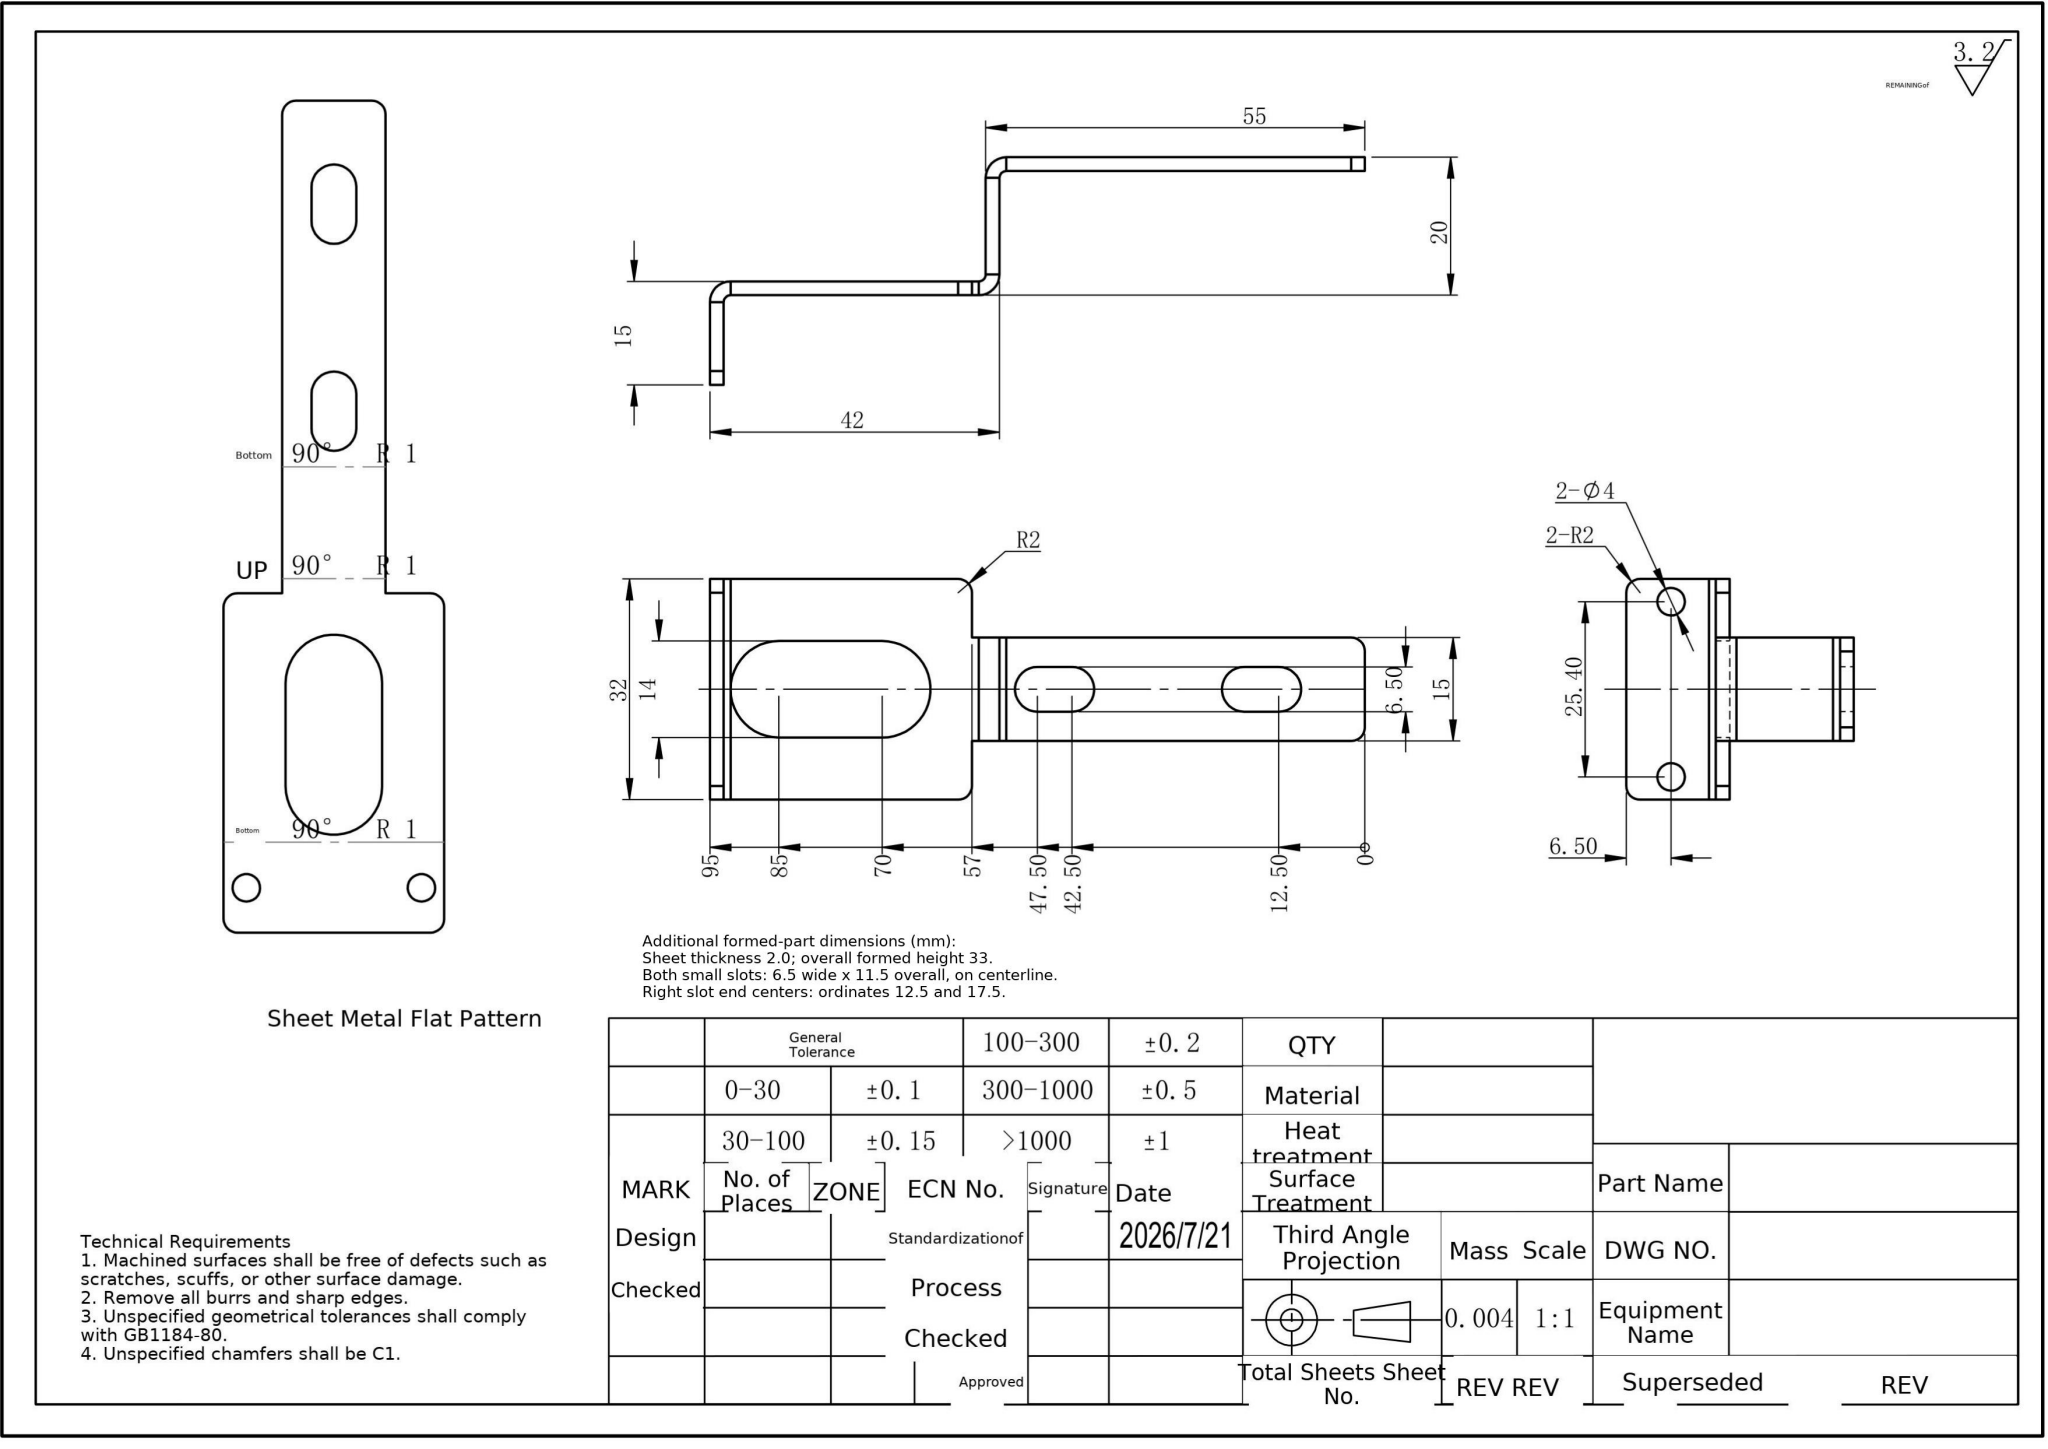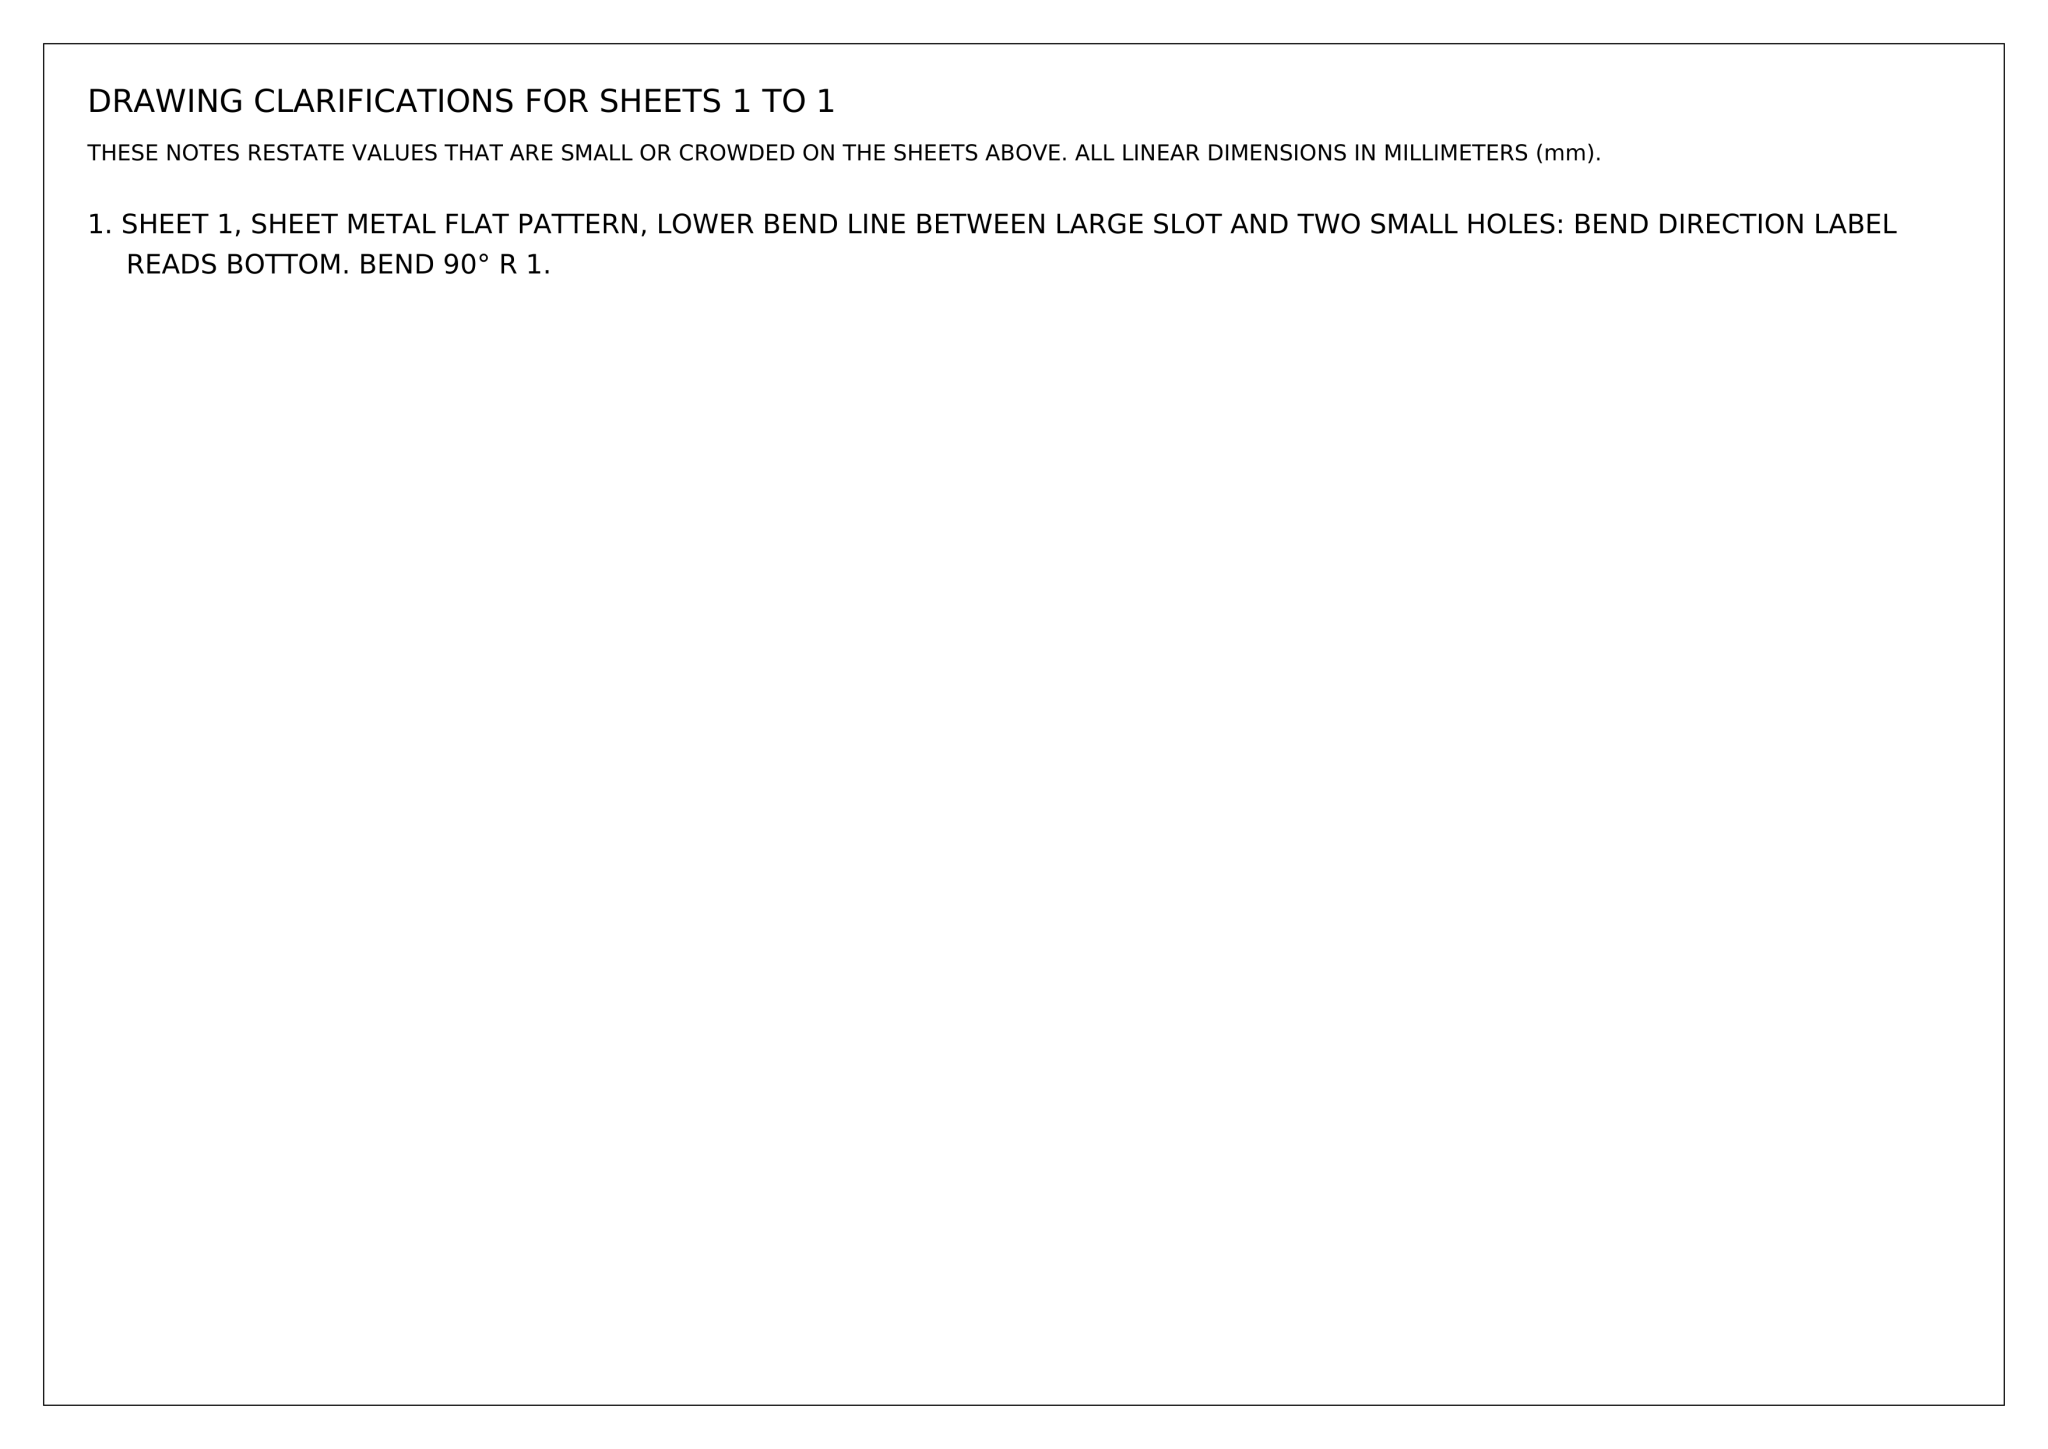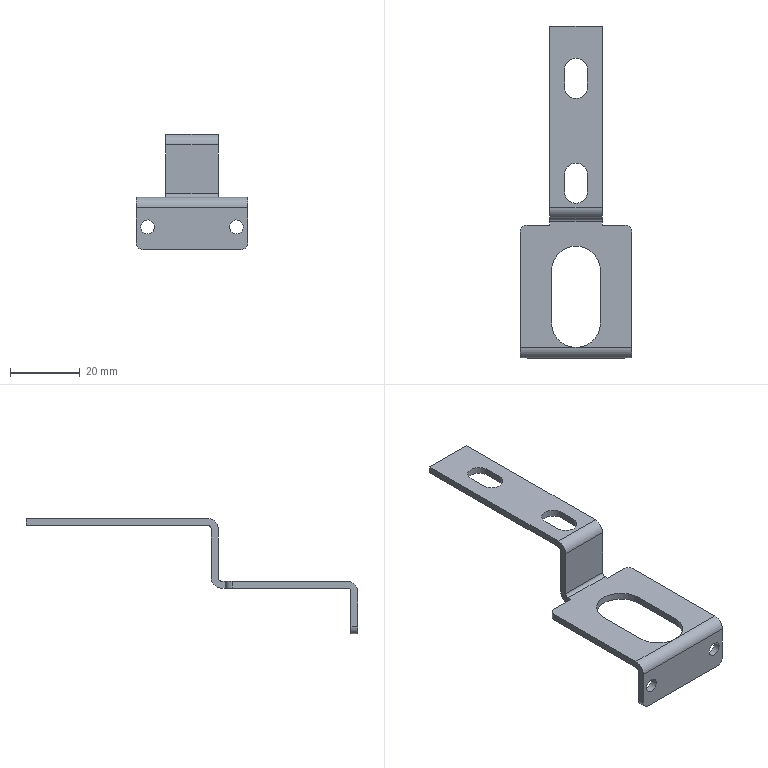Part | NX | mm | Stepped Angled Strap Bracket | 1 solid | 40 faces | box 32 x 95 x 33 mm | volume 4360 mm3 | plane 22 | cylinder 18 | commonest cylinder face diameters 4 x6 6.5 x4 2 x3 6 x3 14 x2